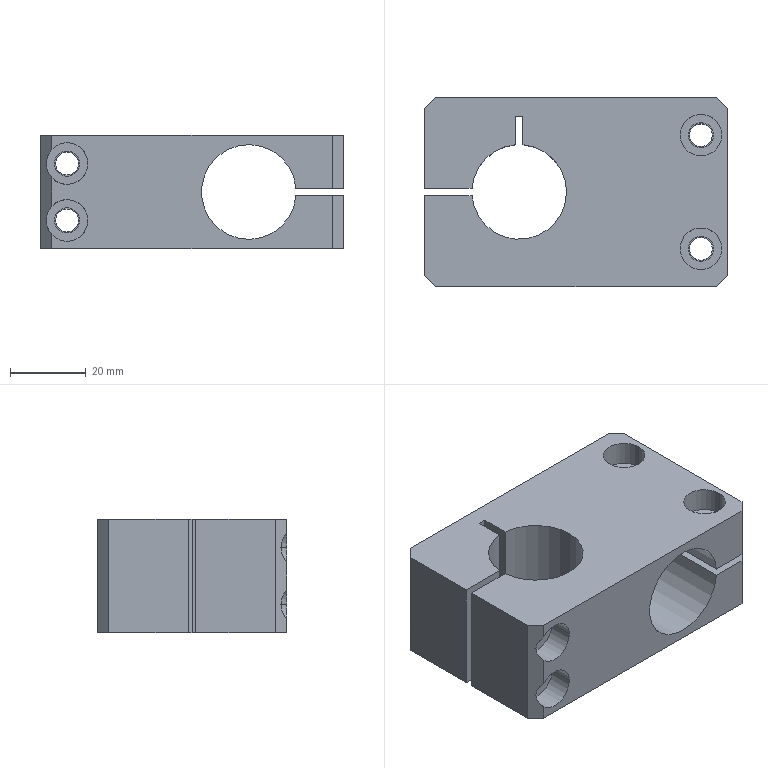Component | SolidWorks | 8TC-A15004-90-03A-1 | 1 solid | 53 faces | box 80 x 50 x 30 mm | volume 71459 mm3 | cylinder 28 | plane 25 | commonest cylinder face diameters 6 x8 11 x8 6.6 x8 25 x4 | material #45
build123d program:
from build123d import *

# Parameters (mm, degrees)
SKETCH1_W                                       = 30
SKETCH1_H                                       = 80
BOSS_EXTRUDE1_DEPTH                             = 25
SKETCH2_R                                       = 12.5
CUT_EXTRUDE1_DEPTH                              = 66.765
SKETCH3_W                                       = 2
SKETCH3_H                                       = 12.54
CUT_EXTRUDE2_DEPTH                              = 66.765
SKETCH4_R                                       = 12.5
CUT_EXTRUDE3_DEPTH                              = 56.902
SKETCH5_W                                       = 12.54
SKETCH5_H                                       = 2
CUT_EXTRUDE4_DEPTH                              = 56.902
SKETCH6_W                                       = 2
SKETCH6_H                                       = 7.54
CUT_EXTRUDE5_DEPTH                              = 56.902
CHAMFER1_SIZE                                   = 3
M6_HEX_SOCKET_HEAD_CAP_SCREW_CBORE1_D           = 6.6
M6_HEX_SOCKET_HEAD_CAP_SCREW_CBORE1_DEPTH       = 14
M6_HEX_SOCKET_HEAD_CAP_SCREW_CBORE1_CBORE_D     = 11
M6_HEX_SOCKET_HEAD_CAP_SCREW_CBORE1_CBORE_DEPTH = 6.4
M6_TAPPED_HOLE1_D                               = 6
M6_HEX_SOCKET_HEAD_CAP_SCREW_CBORE2_D           = 6.6
M6_HEX_SOCKET_HEAD_CAP_SCREW_CBORE2_DEPTH       = 24
M6_HEX_SOCKET_HEAD_CAP_SCREW_CBORE2_CBORE_D     = 11
M6_HEX_SOCKET_HEAD_CAP_SCREW_CBORE2_CBORE_DEPTH = 6.4
M6_TAPPED_HOLE2_D                               = 6


with BuildPart() as part:
    # Sketch1 → Boss-Extrude1 (new, symmetric)
    with BuildSketch(Plane(origin=(0, 0, 0), x_dir=(1, 0, 0), z_dir=(0, 1, 0))):
        Rectangle(SKETCH1_W, SKETCH1_H)
    extrude(amount=BOSS_EXTRUDE1_DEPTH, both=True)

    # Sketch2 → Cut-Extrude1 (cut, through all)
    with BuildSketch(Plane(origin=(0, 25, 0), x_dir=(1, 0, 0), z_dir=(0, 1, 0))):
        with Locations(Location((0, -15, 0), (0, 0, 270))):
            Circle(SKETCH2_R)
    extrude(amount=-CUT_EXTRUDE1_DEPTH, mode=Mode.SUBTRACT)

    # Sketch3 → Cut-Extrude2 (cut, through all)
    with BuildSketch(Plane(origin=(0, 25, 0), x_dir=(1, 0, 0), z_dir=(0, 1, 0))):
        with Locations((0, -33.73)):
            Rectangle(SKETCH3_W, SKETCH3_H)
    extrude(amount=-CUT_EXTRUDE2_DEPTH, mode=Mode.SUBTRACT)

    # Sketch4 → Cut-Extrude3 (cut, through all)
    with BuildSketch(Plane.ZY.offset(15)):
        with Locations((-15, 0)):
            Circle(SKETCH4_R)
    extrude(amount=-CUT_EXTRUDE3_DEPTH, mode=Mode.SUBTRACT)

    # Sketch5 → Cut-Extrude4 (cut, through all)
    with BuildSketch(Plane.ZY.offset(15)):
        with Locations((-33.73, 0)):
            Rectangle(SKETCH5_W, SKETCH5_H)
    extrude(amount=-CUT_EXTRUDE4_DEPTH, mode=Mode.SUBTRACT)

    # Sketch6 → Cut-Extrude5 (cut, through all)
    with BuildSketch(Plane.ZY.offset(15)):
        with Locations((-15, 16.23)):
            Rectangle(SKETCH6_W, SKETCH6_H)
    extrude(amount=-CUT_EXTRUDE5_DEPTH, mode=Mode.SUBTRACT)

    # Chamfer1
    chamfer1_edges = [part.edges().sort_by_distance(p)[0] for p in [
        (-8, 25, 40),
        (8, -25, 40),
        (8, 25, 40),
        (-8, -25, 40),
        (0, -25, -40),
        (0, 25, -40),
    ]]
    chamfer(chamfer1_edges, length=CHAMFER1_SIZE)

    # M6 Hex Socket Head Cap Screw CBORE1
    with Locations(Plane.ZY.offset(15)):
        with Locations((33, 15), (33, -15)):
            CounterBoreHole(M6_HEX_SOCKET_HEAD_CAP_SCREW_CBORE1_D / 2, M6_HEX_SOCKET_HEAD_CAP_SCREW_CBORE1_CBORE_D / 2, M6_HEX_SOCKET_HEAD_CAP_SCREW_CBORE1_CBORE_DEPTH, depth=M6_HEX_SOCKET_HEAD_CAP_SCREW_CBORE1_DEPTH)

    # M6 Tapped Hole1 (through all)
    with Locations(Plane.ZY.offset(-1)):
        with Locations((33, 15), (33, -15)):
            Hole(M6_TAPPED_HOLE1_D / 2)

    # M6 Hex Socket Head Cap Screw CBORE2
    with Locations(Plane(origin=(0, -25, 0), x_dir=(-1, 0, 0), z_dir=(0, -1, 0))):
        with Locations((-7.5, 33), (7.5, 33)):
            CounterBoreHole(M6_HEX_SOCKET_HEAD_CAP_SCREW_CBORE2_D / 2, M6_HEX_SOCKET_HEAD_CAP_SCREW_CBORE2_CBORE_D / 2, M6_HEX_SOCKET_HEAD_CAP_SCREW_CBORE2_CBORE_DEPTH, depth=M6_HEX_SOCKET_HEAD_CAP_SCREW_CBORE2_DEPTH)

    # M6 Tapped Hole2 (through all)
    with Locations(Plane(origin=(0, 1, 0), x_dir=(-1, 0, 0), z_dir=(0, -1, 0))):
        with Locations((-7.5, 33), (7.5, 33)):
            Hole(M6_TAPPED_HOLE2_D / 2)


solid = part.part

# Placed as in the assembly
solid = solid.moved(Location((-30, 329.3, 0), (0, 90, 0)))